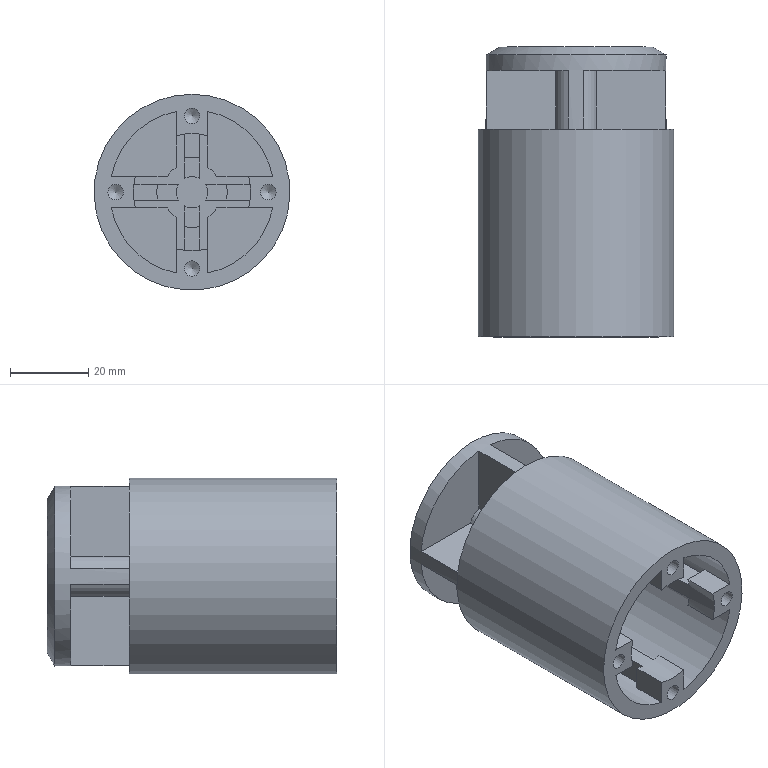Component | NX | VALVE_DISC | 1 solid | 91 faces | volume 57353 mm3 | plane 56 | cylinder 30 | cone 5 | commonest cylinder face diameters 42 x4 18 x4 15 x4 11 x4 30 x4 8 x4 4 x4 46 x1